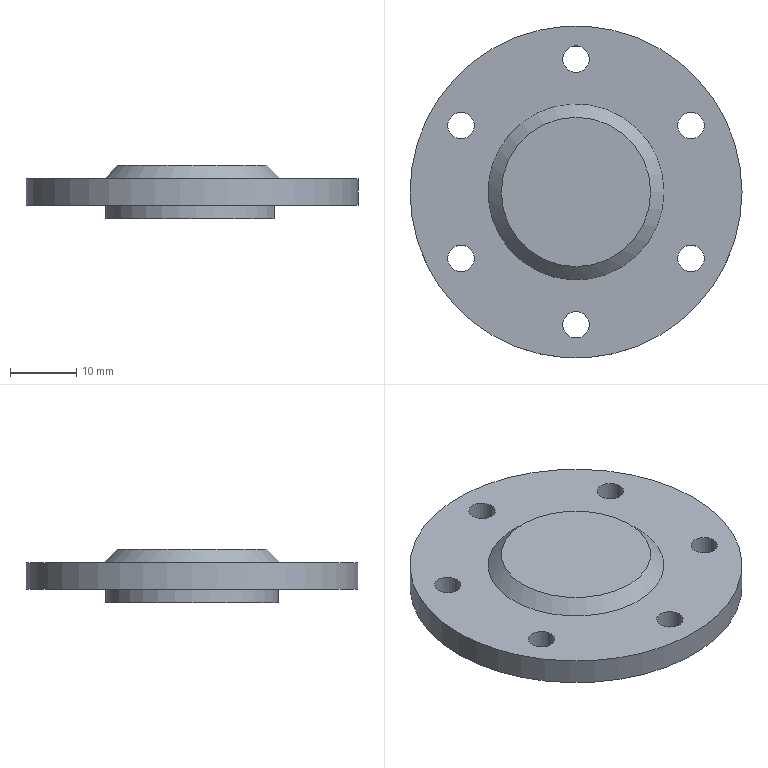Component | NX | 06__27 | 1 solid | 14 faces | box 50 x 50 x 8 mm | volume 9512 mm3 | cylinder 9 | plane 4 | cone 1 | commonest cylinder face diameters 4 x6 50 x1 26 x1 8 x1
STEP:
#1=CARTESIAN_POINT('',(0.,0.,0.));
#2=DIRECTION('',(0.,0.,1.));
#3=DIRECTION('',(1.,0.,0.));
#4=AXIS2_PLACEMENT_3D('',#1,#2,#3);
#5=CARTESIAN_POINT('',(28.272,109.608,238.432));
#6=VERTEX_POINT('',#5);
#7=CARTESIAN_POINT('',(17.022,109.608,238.432));
#8=DIRECTION('',(-0.,0.,1.));
#9=DIRECTION('',(1.,0.,0.));
#10=AXIS2_PLACEMENT_3D('',#7,#8,#9);
#11=CIRCLE('',#10,11.25);
#12=CARTESIAN_POINT('',(17.022,109.608,238.432));
#13=DIRECTION('',(-0.,0.,1.));
#14=DIRECTION('',(1.,0.,0.));
#15=AXIS2_PLACEMENT_3D('',#12,#13,#14);
#16=PLANE('',#15);
#17=CARTESIAN_POINT('',(0.,0.));
#18=DIRECTION('',(1.,0.));
#19=AXIS2_PLACEMENT_2D('',#17,#18);
#20=CIRCLE('',#19,11.25);
#21=(GEOMETRIC_REPRESENTATION_CONTEXT(2)PARAMETRIC_REPRESENTATION_CONTEXT()REPRESENTATION_CONTEXT('',''));
#22=DEFINITIONAL_REPRESENTATION('',(#20),#21);
#23=PCURVE('',#16,#22);
#24=CARTESIAN_POINT('',(17.022,109.608,238.432));
#25=DIRECTION('',(0.,0.,-1.));
#26=DIRECTION('',(-1.,0.,-0.));
#27=AXIS2_PLACEMENT_3D('',#24,#25,#26);
#28=CONICAL_SURFACE('',#27,11.25,0.7854);
#29=CARTESIAN_POINT('',(9.425,0.));
#30=DIRECTION('',(-1.,0.));
#31=VECTOR('',#30,1.);
#32=LINE('',#29,#31);
#33=(GEOMETRIC_REPRESENTATION_CONTEXT(2)PARAMETRIC_REPRESENTATION_CONTEXT()REPRESENTATION_CONTEXT('',''));
#34=DEFINITIONAL_REPRESENTATION('',(#32),#33);
#35=PCURVE('',#28,#34);
#36=SURFACE_CURVE('',#11,(#23,#35),.PCURVE_S1.);
#37=EDGE_CURVE('',#6,#6,#36,.T.);
#38=ORIENTED_EDGE('',*,*,#37,.T.);
#39=EDGE_LOOP('',(#38));
#40=FACE_BOUND('',#39,.T.);
#41=ADVANCED_FACE('',(#40),#16,.T.);
#42=CARTESIAN_POINT('',(30.272,109.608,236.432));
#43=VERTEX_POINT('',#42);
#44=CARTESIAN_POINT('',(17.022,109.608,236.432));
#45=DIRECTION('',(-0.,0.,1.));
#46=DIRECTION('',(1.,0.,0.));
#47=AXIS2_PLACEMENT_3D('',#44,#45,#46);
#48=CIRCLE('',#47,13.25);
#49=CARTESIAN_POINT('',(9.425,2.));
#50=DIRECTION('',(-1.,0.));
#51=VECTOR('',#50,1.);
#52=LINE('',#49,#51);
#53=(GEOMETRIC_REPRESENTATION_CONTEXT(2)PARAMETRIC_REPRESENTATION_CONTEXT()REPRESENTATION_CONTEXT('',''));
#54=DEFINITIONAL_REPRESENTATION('',(#52),#53);
#55=PCURVE('',#28,#54);
#56=CARTESIAN_POINT('',(30.272,109.608,236.432));
#57=DIRECTION('',(-0.,0.,1.));
#58=DIRECTION('',(1.,0.,0.));
#59=AXIS2_PLACEMENT_3D('',#56,#57,#58);
#60=PLANE('',#59);
#61=CARTESIAN_POINT('',(-13.25,0.));
#62=DIRECTION('',(1.,0.));
#63=AXIS2_PLACEMENT_2D('',#61,#62);
#64=CIRCLE('',#63,13.25);
#65=(GEOMETRIC_REPRESENTATION_CONTEXT(2)PARAMETRIC_REPRESENTATION_CONTEXT()REPRESENTATION_CONTEXT('',''));
#66=DEFINITIONAL_REPRESENTATION('',(#64),#65);
#67=PCURVE('',#60,#66);
#68=SURFACE_CURVE('',#48,(#55,#67),.PCURVE_S1.);
#69=EDGE_CURVE('',#43,#43,#68,.T.);
#70=ORIENTED_EDGE('',*,*,#69,.T.);
#71=CARTESIAN_POINT('',(28.272,109.608,238.432));
#72=CARTESIAN_POINT('',(30.272,109.608,236.432));
#73=B_SPLINE_CURVE_WITH_KNOTS('',1,(#71,#72),.UNSPECIFIED.,.F.,.F.,(2,2),(0.,2.828),.PIECEWISE_BEZIER_KNOTS.);
#74=CARTESIAN_POINT('',(3.142,0.));
#75=DIRECTION('',(0.,1.));
#76=VECTOR('',#75,1.);
#77=LINE('',#74,#76);
#78=(GEOMETRIC_REPRESENTATION_CONTEXT(2)PARAMETRIC_REPRESENTATION_CONTEXT()REPRESENTATION_CONTEXT('',''));
#79=DEFINITIONAL_REPRESENTATION('',(#77),#78);
#80=PCURVE('',#28,#79);
#81=CARTESIAN_POINT('',(9.425,0.));
#82=DIRECTION('',(0.,1.));
#83=VECTOR('',#82,1.);
#84=LINE('',#81,#83);
#85=(GEOMETRIC_REPRESENTATION_CONTEXT(2)PARAMETRIC_REPRESENTATION_CONTEXT()REPRESENTATION_CONTEXT('',''));
#86=DEFINITIONAL_REPRESENTATION('',(#84),#85);
#87=PCURVE('',#28,#86);
#88=SEAM_CURVE('',#73,(#80,#87),.PCURVE_S1.);
#89=EDGE_CURVE('',#6,#43,#88,.T.);
#90=ORIENTED_EDGE('',*,*,#89,.F.);
#91=ORIENTED_EDGE('',*,*,#37,.F.);
#92=ORIENTED_EDGE('',*,*,#89,.T.);
#93=EDGE_LOOP('',(#70,#90,#91,#92));
#94=FACE_BOUND('',#93,.T.);
#95=ADVANCED_FACE('',(#94),#28,.T.);
#96=CARTESIAN_POINT('',(19.022,129.608,236.432));
#97=VERTEX_POINT('',#96);
#98=CARTESIAN_POINT('',(17.022,129.608,236.432));
#99=DIRECTION('',(-0.,0.,1.));
#100=DIRECTION('',(1.,0.,0.));
#101=AXIS2_PLACEMENT_3D('',#98,#99,#100);
#102=CIRCLE('',#101,2.);
#103=CARTESIAN_POINT('',(-13.25,20.));
#104=DIRECTION('',(1.,0.));
#105=AXIS2_PLACEMENT_2D('',#103,#104);
#106=CIRCLE('',#105,2.);
#107=(GEOMETRIC_REPRESENTATION_CONTEXT(2)PARAMETRIC_REPRESENTATION_CONTEXT()REPRESENTATION_CONTEXT('',''));
#108=DEFINITIONAL_REPRESENTATION('',(#106),#107);
#109=PCURVE('',#60,#108);
#110=CARTESIAN_POINT('',(17.022,129.608,248.732));
#111=DIRECTION('',(0.,0.,-1.));
#112=DIRECTION('',(0.,1.,0.));
#113=AXIS2_PLACEMENT_3D('',#110,#111,#112);
#114=CYLINDRICAL_SURFACE('',#113,2.);
#115=CARTESIAN_POINT('',(7.854,12.3));
#116=DIRECTION('',(-1.,0.));
#117=VECTOR('',#116,1.);
#118=LINE('',#115,#117);
#119=(GEOMETRIC_REPRESENTATION_CONTEXT(2)PARAMETRIC_REPRESENTATION_CONTEXT()REPRESENTATION_CONTEXT('',''));
#120=DEFINITIONAL_REPRESENTATION('',(#118),#119);
#121=PCURVE('',#114,#120);
#122=SURFACE_CURVE('',#102,(#109,#121),.PCURVE_S1.);
#123=EDGE_CURVE('',#97,#97,#122,.T.);
#124=ORIENTED_EDGE('',*,*,#123,.F.);
#125=EDGE_LOOP('',(#124));
#126=FACE_BOUND('',#125,.T.);
#127=CARTESIAN_POINT('',(36.343,119.608,236.432));
#128=VERTEX_POINT('',#127);
#129=CARTESIAN_POINT('',(34.343,119.608,236.432));
#130=DIRECTION('',(-0.,0.,1.));
#131=DIRECTION('',(1.,0.,0.));
#132=AXIS2_PLACEMENT_3D('',#129,#130,#131);
#133=CIRCLE('',#132,2.);
#134=CARTESIAN_POINT('',(4.071,10.));
#135=DIRECTION('',(1.,0.));
#136=AXIS2_PLACEMENT_2D('',#134,#135);
#137=CIRCLE('',#136,2.);
#138=(GEOMETRIC_REPRESENTATION_CONTEXT(2)PARAMETRIC_REPRESENTATION_CONTEXT()REPRESENTATION_CONTEXT('',''));
#139=DEFINITIONAL_REPRESENTATION('',(#137),#138);
#140=PCURVE('',#60,#139);
#141=CARTESIAN_POINT('',(34.343,119.608,248.732));
#142=DIRECTION('',(0.,0.,-1.));
#143=DIRECTION('',(0.,1.,0.));
#144=AXIS2_PLACEMENT_3D('',#141,#142,#143);
#145=CYLINDRICAL_SURFACE('',#144,2.);
#146=CARTESIAN_POINT('',(7.854,12.3));
#147=DIRECTION('',(-1.,0.));
#148=VECTOR('',#147,1.);
#149=LINE('',#146,#148);
#150=(GEOMETRIC_REPRESENTATION_CONTEXT(2)PARAMETRIC_REPRESENTATION_CONTEXT()REPRESENTATION_CONTEXT('',''));
#151=DEFINITIONAL_REPRESENTATION('',(#149),#150);
#152=PCURVE('',#145,#151);
#153=SURFACE_CURVE('',#133,(#140,#152),.PCURVE_S1.);
#154=EDGE_CURVE('',#128,#128,#153,.T.);
#155=ORIENTED_EDGE('',*,*,#154,.F.);
#156=EDGE_LOOP('',(#155));
#157=FACE_BOUND('',#156,.T.);
#158=CARTESIAN_POINT('',(1.702,119.608,236.432));
#159=VERTEX_POINT('',#158);
#160=CARTESIAN_POINT('',(-0.2984,119.608,236.432));
#161=DIRECTION('',(-0.,0.,1.));
#162=DIRECTION('',(1.,0.,0.));
#163=AXIS2_PLACEMENT_3D('',#160,#161,#162);
#164=CIRCLE('',#163,2.);
#165=CARTESIAN_POINT('',(-30.571,10.));
#166=DIRECTION('',(1.,0.));
#167=AXIS2_PLACEMENT_2D('',#165,#166);
#168=CIRCLE('',#167,2.);
#169=(GEOMETRIC_REPRESENTATION_CONTEXT(2)PARAMETRIC_REPRESENTATION_CONTEXT()REPRESENTATION_CONTEXT('',''));
#170=DEFINITIONAL_REPRESENTATION('',(#168),#169);
#171=PCURVE('',#60,#170);
#172=CARTESIAN_POINT('',(-0.2984,119.608,248.732));
#173=DIRECTION('',(0.,0.,-1.));
#174=DIRECTION('',(0.,1.,0.));
#175=AXIS2_PLACEMENT_3D('',#172,#173,#174);
#176=CYLINDRICAL_SURFACE('',#175,2.);
#177=CARTESIAN_POINT('',(7.854,12.3));
#178=DIRECTION('',(-1.,0.));
#179=VECTOR('',#178,1.);
#180=LINE('',#177,#179);
#181=(GEOMETRIC_REPRESENTATION_CONTEXT(2)PARAMETRIC_REPRESENTATION_CONTEXT()REPRESENTATION_CONTEXT('',''));
#182=DEFINITIONAL_REPRESENTATION('',(#180),#181);
#183=PCURVE('',#176,#182);
#184=SURFACE_CURVE('',#164,(#171,#183),.PCURVE_S1.);
#185=EDGE_CURVE('',#159,#159,#184,.T.);
#186=ORIENTED_EDGE('',*,*,#185,.F.);
#187=EDGE_LOOP('',(#186));
#188=FACE_BOUND('',#187,.T.);
#189=CARTESIAN_POINT('',(36.343,99.608,236.432));
#190=VERTEX_POINT('',#189);
#191=CARTESIAN_POINT('',(34.343,99.608,236.432));
#192=DIRECTION('',(-0.,0.,1.));
#193=DIRECTION('',(1.,0.,0.));
#194=AXIS2_PLACEMENT_3D('',#191,#192,#193);
#195=CIRCLE('',#194,2.);
#196=CARTESIAN_POINT('',(4.071,-10.));
#197=DIRECTION('',(1.,0.));
#198=AXIS2_PLACEMENT_2D('',#196,#197);
#199=CIRCLE('',#198,2.);
#200=(GEOMETRIC_REPRESENTATION_CONTEXT(2)PARAMETRIC_REPRESENTATION_CONTEXT()REPRESENTATION_CONTEXT('',''));
#201=DEFINITIONAL_REPRESENTATION('',(#199),#200);
#202=PCURVE('',#60,#201);
#203=CARTESIAN_POINT('',(34.343,99.608,248.732));
#204=DIRECTION('',(0.,0.,-1.));
#205=DIRECTION('',(0.,1.,0.));
#206=AXIS2_PLACEMENT_3D('',#203,#204,#205);
#207=CYLINDRICAL_SURFACE('',#206,2.);
#208=CARTESIAN_POINT('',(7.854,12.3));
#209=DIRECTION('',(-1.,0.));
#210=VECTOR('',#209,1.);
#211=LINE('',#208,#210);
#212=(GEOMETRIC_REPRESENTATION_CONTEXT(2)PARAMETRIC_REPRESENTATION_CONTEXT()REPRESENTATION_CONTEXT('',''));
#213=DEFINITIONAL_REPRESENTATION('',(#211),#212);
#214=PCURVE('',#207,#213);
#215=SURFACE_CURVE('',#195,(#202,#214),.PCURVE_S1.);
#216=EDGE_CURVE('',#190,#190,#215,.T.);
#217=ORIENTED_EDGE('',*,*,#216,.F.);
#218=EDGE_LOOP('',(#217));
#219=FACE_BOUND('',#218,.T.);
#220=CARTESIAN_POINT('',(1.702,99.608,236.432));
#221=VERTEX_POINT('',#220);
#222=CARTESIAN_POINT('',(-0.2984,99.608,236.432));
#223=DIRECTION('',(-0.,0.,1.));
#224=DIRECTION('',(1.,0.,0.));
#225=AXIS2_PLACEMENT_3D('',#222,#223,#224);
#226=CIRCLE('',#225,2.);
#227=CARTESIAN_POINT('',(-30.571,-10.));
#228=DIRECTION('',(1.,0.));
#229=AXIS2_PLACEMENT_2D('',#227,#228);
#230=CIRCLE('',#229,2.);
#231=(GEOMETRIC_REPRESENTATION_CONTEXT(2)PARAMETRIC_REPRESENTATION_CONTEXT()REPRESENTATION_CONTEXT('',''));
#232=DEFINITIONAL_REPRESENTATION('',(#230),#231);
#233=PCURVE('',#60,#232);
#234=CARTESIAN_POINT('',(-0.2984,99.608,248.732));
#235=DIRECTION('',(0.,0.,-1.));
#236=DIRECTION('',(0.,1.,0.));
#237=AXIS2_PLACEMENT_3D('',#234,#235,#236);
#238=CYLINDRICAL_SURFACE('',#237,2.);
#239=CARTESIAN_POINT('',(7.854,12.3));
#240=DIRECTION('',(-1.,0.));
#241=VECTOR('',#240,1.);
#242=LINE('',#239,#241);
#243=(GEOMETRIC_REPRESENTATION_CONTEXT(2)PARAMETRIC_REPRESENTATION_CONTEXT()REPRESENTATION_CONTEXT('',''));
#244=DEFINITIONAL_REPRESENTATION('',(#242),#243);
#245=PCURVE('',#238,#244);
#246=SURFACE_CURVE('',#226,(#233,#245),.PCURVE_S1.);
#247=EDGE_CURVE('',#221,#221,#246,.T.);
#248=ORIENTED_EDGE('',*,*,#247,.F.);
#249=EDGE_LOOP('',(#248));
#250=FACE_BOUND('',#249,.T.);
#251=CARTESIAN_POINT('',(19.022,89.608,236.432));
#252=VERTEX_POINT('',#251);
#253=CARTESIAN_POINT('',(17.022,89.608,236.432));
#254=DIRECTION('',(-0.,0.,1.));
#255=DIRECTION('',(1.,0.,0.));
#256=AXIS2_PLACEMENT_3D('',#253,#254,#255);
#257=CIRCLE('',#256,2.);
#258=CARTESIAN_POINT('',(-13.25,-20.));
#259=DIRECTION('',(1.,0.));
#260=AXIS2_PLACEMENT_2D('',#258,#259);
#261=CIRCLE('',#260,2.);
#262=(GEOMETRIC_REPRESENTATION_CONTEXT(2)PARAMETRIC_REPRESENTATION_CONTEXT()REPRESENTATION_CONTEXT('',''));
#263=DEFINITIONAL_REPRESENTATION('',(#261),#262);
#264=PCURVE('',#60,#263);
#265=CARTESIAN_POINT('',(17.022,89.608,248.732));
#266=DIRECTION('',(0.,0.,-1.));
#267=DIRECTION('',(0.,1.,0.));
#268=AXIS2_PLACEMENT_3D('',#265,#266,#267);
#269=CYLINDRICAL_SURFACE('',#268,2.);
#270=CARTESIAN_POINT('',(7.854,12.3));
#271=DIRECTION('',(-1.,0.));
#272=VECTOR('',#271,1.);
#273=LINE('',#270,#272);
#274=(GEOMETRIC_REPRESENTATION_CONTEXT(2)PARAMETRIC_REPRESENTATION_CONTEXT()REPRESENTATION_CONTEXT('',''));
#275=DEFINITIONAL_REPRESENTATION('',(#273),#274);
#276=PCURVE('',#269,#275);
#277=SURFACE_CURVE('',#257,(#264,#276),.PCURVE_S1.);
#278=EDGE_CURVE('',#252,#252,#277,.T.);
#279=ORIENTED_EDGE('',*,*,#278,.F.);
#280=EDGE_LOOP('',(#279));
#281=FACE_BOUND('',#280,.T.);
#282=CARTESIAN_POINT('',(42.022,109.608,236.432));
#283=VERTEX_POINT('',#282);
#284=CARTESIAN_POINT('',(17.022,109.608,236.432));
#285=DIRECTION('',(-0.,0.,1.));
#286=DIRECTION('',(1.,0.,0.));
#287=AXIS2_PLACEMENT_3D('',#284,#285,#286);
#288=CIRCLE('',#287,25.);
#289=CARTESIAN_POINT('',(-13.25,0.));
#290=DIRECTION('',(1.,0.));
#291=AXIS2_PLACEMENT_2D('',#289,#290);
#292=CIRCLE('',#291,25.);
#293=(GEOMETRIC_REPRESENTATION_CONTEXT(2)PARAMETRIC_REPRESENTATION_CONTEXT()REPRESENTATION_CONTEXT('',''));
#294=DEFINITIONAL_REPRESENTATION('',(#292),#293);
#295=PCURVE('',#60,#294);
#296=CARTESIAN_POINT('',(17.022,109.608,230.432));
#297=DIRECTION('',(-0.,0.,1.));
#298=DIRECTION('',(1.,0.,0.));
#299=AXIS2_PLACEMENT_3D('',#296,#297,#298);
#300=CYLINDRICAL_SURFACE('',#299,25.);
#301=CARTESIAN_POINT('',(0.,6.));
#302=DIRECTION('',(1.,0.));
#303=VECTOR('',#302,1.);
#304=LINE('',#301,#303);
#305=(GEOMETRIC_REPRESENTATION_CONTEXT(2)PARAMETRIC_REPRESENTATION_CONTEXT()REPRESENTATION_CONTEXT('',''));
#306=DEFINITIONAL_REPRESENTATION('',(#304),#305);
#307=PCURVE('',#300,#306);
#308=SURFACE_CURVE('',#288,(#295,#307),.PCURVE_S1.);
#309=EDGE_CURVE('',#283,#283,#308,.T.);
#310=ORIENTED_EDGE('',*,*,#309,.T.);
#311=EDGE_LOOP('',(#310));
#312=FACE_BOUND('',#311,.T.);
#313=ORIENTED_EDGE('',*,*,#69,.F.);
#314=EDGE_LOOP('',(#313));
#315=FACE_BOUND('',#314,.T.);
#316=ADVANCED_FACE('',(#126,#157,#188,#219,#250,#281,#312,#315),#60,.T.);
#317=CARTESIAN_POINT('',(42.022,109.608,232.432));
#318=VERTEX_POINT('',#317);
#319=CARTESIAN_POINT('',(17.022,109.608,232.432));
#320=DIRECTION('',(-0.,0.,1.));
#321=DIRECTION('',(1.,0.,0.));
#322=AXIS2_PLACEMENT_3D('',#319,#320,#321);
#323=CIRCLE('',#322,25.);
#324=CARTESIAN_POINT('',(0.,2.));
#325=DIRECTION('',(1.,0.));
#326=VECTOR('',#325,1.);
#327=LINE('',#324,#326);
#328=(GEOMETRIC_REPRESENTATION_CONTEXT(2)PARAMETRIC_REPRESENTATION_CONTEXT()REPRESENTATION_CONTEXT('',''));
#329=DEFINITIONAL_REPRESENTATION('',(#327),#328);
#330=PCURVE('',#300,#329);
#331=CARTESIAN_POINT('',(42.022,109.608,232.432));
#332=DIRECTION('',(0.,0.,-1.));
#333=DIRECTION('',(-1.,0.,-0.));
#334=AXIS2_PLACEMENT_3D('',#331,#332,#333);
#335=PLANE('',#334);
#336=CARTESIAN_POINT('',(0.,0.));
#337=CARTESIAN_POINT('',(0.,43.301));
#338=CARTESIAN_POINT('',(37.5,21.651));
#339=CARTESIAN_POINT('',(75.,0.));
#340=CARTESIAN_POINT('',(37.5,-21.651));
#341=CARTESIAN_POINT('',(0.,-43.301));
#342=CARTESIAN_POINT('',(0.,0.));
#343=(BOUNDED_CURVE()B_SPLINE_CURVE(2,(#336,#337,#338,#339,#340,#341,#342),.UNSPECIFIED.,.T.,.F.)B_SPLINE_CURVE_WITH_KNOTS((1,2,2,2,2,1),(-2.094,0.,2.094,4.189,6.283,8.378),.UNSPECIFIED.)CURVE()GEOMETRIC_REPRESENTATION_ITEM()RATIONAL_B_SPLINE_CURVE((1.,0.5,1.,0.5,1.,0.5,1.))REPRESENTATION_ITEM(''));
#344=(GEOMETRIC_REPRESENTATION_CONTEXT(2)PARAMETRIC_REPRESENTATION_CONTEXT()REPRESENTATION_CONTEXT('',''));
#345=DEFINITIONAL_REPRESENTATION('',(#343),#344);
#346=PCURVE('',#335,#345);
#347=SURFACE_CURVE('',#323,(#330,#346),.PCURVE_S1.);
#348=EDGE_CURVE('',#318,#318,#347,.T.);
#349=ORIENTED_EDGE('',*,*,#348,.T.);
#350=CARTESIAN_POINT('',(42.022,109.608,232.432));
#351=CARTESIAN_POINT('',(42.022,109.608,236.432));
#352=B_SPLINE_CURVE_WITH_KNOTS('',1,(#350,#351),.UNSPECIFIED.,.F.,.F.,(2,2),(2.,6.),.PIECEWISE_BEZIER_KNOTS.);
#353=CARTESIAN_POINT('',(6.283,0.));
#354=DIRECTION('',(0.,1.));
#355=VECTOR('',#354,1.);
#356=LINE('',#353,#355);
#357=(GEOMETRIC_REPRESENTATION_CONTEXT(2)PARAMETRIC_REPRESENTATION_CONTEXT()REPRESENTATION_CONTEXT('',''));
#358=DEFINITIONAL_REPRESENTATION('',(#356),#357);
#359=PCURVE('',#300,#358);
#360=CARTESIAN_POINT('',(0.,0.));
#361=DIRECTION('',(0.,1.));
#362=VECTOR('',#361,1.);
#363=LINE('',#360,#362);
#364=(GEOMETRIC_REPRESENTATION_CONTEXT(2)PARAMETRIC_REPRESENTATION_CONTEXT()REPRESENTATION_CONTEXT('',''));
#365=DEFINITIONAL_REPRESENTATION('',(#363),#364);
#366=PCURVE('',#300,#365);
#367=SEAM_CURVE('',#352,(#359,#366),.PCURVE_S1.);
#368=EDGE_CURVE('',#318,#283,#367,.T.);
#369=ORIENTED_EDGE('',*,*,#368,.T.);
#370=ORIENTED_EDGE('',*,*,#309,.F.);
#371=ORIENTED_EDGE('',*,*,#368,.F.);
#372=EDGE_LOOP('',(#349,#369,#370,#371));
#373=FACE_BOUND('',#372,.T.);
#374=ADVANCED_FACE('',(#373),#300,.T.);
#375=CARTESIAN_POINT('',(29.407,113.56,232.432));
#376=VERTEX_POINT('',#375);
#377=CARTESIAN_POINT('',(29.407,105.656,232.432));
#378=VERTEX_POINT('',#377);
#379=CARTESIAN_POINT('',(17.022,109.608,232.432));
#380=DIRECTION('',(-0.,0.,1.));
#381=DIRECTION('',(1.,0.,0.));
#382=AXIS2_PLACEMENT_3D('',#379,#380,#381);
#383=CIRCLE('',#382,13.);
#384=CARTESIAN_POINT('',(12.,0.));
#385=CARTESIAN_POINT('',(12.,22.517));
#386=CARTESIAN_POINT('',(31.5,11.258));
#387=CARTESIAN_POINT('',(51.,0.));
#388=CARTESIAN_POINT('',(31.5,-11.258));
#389=CARTESIAN_POINT('',(12.,-22.517));
#390=CARTESIAN_POINT('',(12.,0.));
#391=(BOUNDED_CURVE()B_SPLINE_CURVE(2,(#384,#385,#386,#387,#388,#389,#390),.UNSPECIFIED.,.T.,.F.)B_SPLINE_CURVE_WITH_KNOTS((1,2,2,2,2,1),(-2.094,0.,2.094,4.189,6.283,8.378),.UNSPECIFIED.)CURVE()GEOMETRIC_REPRESENTATION_ITEM()RATIONAL_B_SPLINE_CURVE((1.,0.5,1.,0.5,1.,0.5,1.))REPRESENTATION_ITEM(''));
#392=(GEOMETRIC_REPRESENTATION_CONTEXT(2)PARAMETRIC_REPRESENTATION_CONTEXT()REPRESENTATION_CONTEXT('',''));
#393=DEFINITIONAL_REPRESENTATION('',(#391),#392);
#394=PCURVE('',#335,#393);
#395=CARTESIAN_POINT('',(17.022,109.608,230.432));
#396=DIRECTION('',(-0.,0.,1.));
#397=DIRECTION('',(1.,0.,0.));
#398=AXIS2_PLACEMENT_3D('',#395,#396,#397);
#399=CYLINDRICAL_SURFACE('',#398,13.);
#400=CARTESIAN_POINT('',(-0.,2.));
#401=DIRECTION('',(1.,0.));
#402=VECTOR('',#401,1.);
#403=LINE('',#400,#402);
#404=(GEOMETRIC_REPRESENTATION_CONTEXT(2)PARAMETRIC_REPRESENTATION_CONTEXT()REPRESENTATION_CONTEXT('',''));
#405=DEFINITIONAL_REPRESENTATION('',(#403),#404);
#406=PCURVE('',#399,#405);
#407=SURFACE_CURVE('',#383,(#394,#406),.PCURVE_S1.);
#408=EDGE_CURVE('',#376,#378,#407,.T.);
#409=ORIENTED_EDGE('',*,*,#408,.T.);
#410=CARTESIAN_POINT('',(30.022,109.608,232.432));
#411=DIRECTION('',(0.,0.,-1.));
#412=DIRECTION('',(0.,1.,0.));
#413=AXIS2_PLACEMENT_3D('',#410,#411,#412);
#414=CIRCLE('',#413,4.);
#415=CARTESIAN_POINT('',(12.,0.));
#416=DIRECTION('',(0.,1.));
#417=AXIS2_PLACEMENT_2D('',#415,#416);
#418=CIRCLE('',#417,4.);
#419=(GEOMETRIC_REPRESENTATION_CONTEXT(2)PARAMETRIC_REPRESENTATION_CONTEXT()REPRESENTATION_CONTEXT('',''));
#420=DEFINITIONAL_REPRESENTATION('',(#418),#419);
#421=PCURVE('',#335,#420);
#422=CARTESIAN_POINT('',(30.022,109.608,232.432));
#423=DIRECTION('',(0.,0.,-1.));
#424=DIRECTION('',(0.,1.,0.));
#425=AXIS2_PLACEMENT_3D('',#422,#423,#424);
#426=CYLINDRICAL_SURFACE('',#425,4.);
#427=CARTESIAN_POINT('',(-0.,0.));
#428=DIRECTION('',(1.,0.));
#429=VECTOR('',#428,1.);
#430=LINE('',#427,#429);
#431=(GEOMETRIC_REPRESENTATION_CONTEXT(2)PARAMETRIC_REPRESENTATION_CONTEXT()REPRESENTATION_CONTEXT('',''));
#432=DEFINITIONAL_REPRESENTATION('',(#430),#431);
#433=PCURVE('',#426,#432);
#434=SURFACE_CURVE('',#414,(#421,#433),.PCURVE_S1.);
#435=EDGE_CURVE('',#378,#376,#434,.T.);
#436=ORIENTED_EDGE('',*,*,#435,.T.);
#437=EDGE_LOOP('',(#409,#436));
#438=FACE_BOUND('',#437,.T.);
#439=CARTESIAN_POINT('',(15.022,129.608,232.432));
#440=VERTEX_POINT('',#439);
#441=CARTESIAN_POINT('',(19.022,129.608,232.432));
#442=VERTEX_POINT('',#441);
#443=CARTESIAN_POINT('',(17.022,129.608,232.432));
#444=DIRECTION('',(0.,0.,-1.));
#445=DIRECTION('',(-1.,0.,-0.));
#446=AXIS2_PLACEMENT_3D('',#443,#444,#445);
#447=CIRCLE('',#446,2.);
#448=CARTESIAN_POINT('',(25.,20.));
#449=DIRECTION('',(1.,0.));
#450=AXIS2_PLACEMENT_2D('',#448,#449);
#451=CIRCLE('',#450,2.);
#452=(GEOMETRIC_REPRESENTATION_CONTEXT(2)PARAMETRIC_REPRESENTATION_CONTEXT()REPRESENTATION_CONTEXT('',''));
#453=DEFINITIONAL_REPRESENTATION('',(#451),#452);
#454=PCURVE('',#335,#453);
#455=CARTESIAN_POINT('',(4.712,16.3));
#456=DIRECTION('',(1.,0.));
#457=VECTOR('',#456,1.);
#458=LINE('',#455,#457);
#459=(GEOMETRIC_REPRESENTATION_CONTEXT(2)PARAMETRIC_REPRESENTATION_CONTEXT()REPRESENTATION_CONTEXT('',''));
#460=DEFINITIONAL_REPRESENTATION('',(#458),#459);
#461=PCURVE('',#114,#460);
#462=SURFACE_CURVE('',#447,(#454,#461),.PCURVE_S1.);
#463=EDGE_CURVE('',#440,#442,#462,.T.);
#464=ORIENTED_EDGE('',*,*,#463,.F.);
#465=CARTESIAN_POINT('',(17.022,129.608,232.432));
#466=DIRECTION('',(0.,0.,-1.));
#467=DIRECTION('',(-1.,0.,-0.));
#468=AXIS2_PLACEMENT_3D('',#465,#466,#467);
#469=CIRCLE('',#468,2.);
#470=CARTESIAN_POINT('',(25.,20.));
#471=DIRECTION('',(1.,0.));
#472=AXIS2_PLACEMENT_2D('',#470,#471);
#473=CIRCLE('',#472,2.);
#474=(GEOMETRIC_REPRESENTATION_CONTEXT(2)PARAMETRIC_REPRESENTATION_CONTEXT()REPRESENTATION_CONTEXT('',''));
#475=DEFINITIONAL_REPRESENTATION('',(#473),#474);
#476=PCURVE('',#335,#475);
#477=CARTESIAN_POINT('',(-1.571,16.3));
#478=DIRECTION('',(1.,0.));
#479=VECTOR('',#478,1.);
#480=LINE('',#477,#479);
#481=(GEOMETRIC_REPRESENTATION_CONTEXT(2)PARAMETRIC_REPRESENTATION_CONTEXT()REPRESENTATION_CONTEXT('',''));
#482=DEFINITIONAL_REPRESENTATION('',(#480),#481);
#483=PCURVE('',#114,#482);
#484=SURFACE_CURVE('',#469,(#476,#483),.PCURVE_S1.);
#485=EDGE_CURVE('',#442,#440,#484,.T.);
#486=ORIENTED_EDGE('',*,*,#485,.F.);
#487=EDGE_LOOP('',(#464,#486));
#488=FACE_BOUND('',#487,.T.);
#489=CARTESIAN_POINT('',(32.343,119.608,232.432));
#490=VERTEX_POINT('',#489);
#491=CARTESIAN_POINT('',(36.343,119.608,232.432));
#492=VERTEX_POINT('',#491);
#493=CARTESIAN_POINT('',(34.343,119.608,232.432));
#494=DIRECTION('',(0.,0.,-1.));
#495=DIRECTION('',(-1.,0.,-0.));
#496=AXIS2_PLACEMENT_3D('',#493,#494,#495);
#497=CIRCLE('',#496,2.);
#498=CARTESIAN_POINT('',(7.679,10.));
#499=DIRECTION('',(1.,0.));
#500=AXIS2_PLACEMENT_2D('',#498,#499);
#501=CIRCLE('',#500,2.);
#502=(GEOMETRIC_REPRESENTATION_CONTEXT(2)PARAMETRIC_REPRESENTATION_CONTEXT()REPRESENTATION_CONTEXT('',''));
#503=DEFINITIONAL_REPRESENTATION('',(#501),#502);
#504=PCURVE('',#335,#503);
#505=CARTESIAN_POINT('',(4.712,16.3));
#506=DIRECTION('',(1.,0.));
#507=VECTOR('',#506,1.);
#508=LINE('',#505,#507);
#509=(GEOMETRIC_REPRESENTATION_CONTEXT(2)PARAMETRIC_REPRESENTATION_CONTEXT()REPRESENTATION_CONTEXT('',''));
#510=DEFINITIONAL_REPRESENTATION('',(#508),#509);
#511=PCURVE('',#145,#510);
#512=SURFACE_CURVE('',#497,(#504,#511),.PCURVE_S1.);
#513=EDGE_CURVE('',#490,#492,#512,.T.);
#514=ORIENTED_EDGE('',*,*,#513,.F.);
#515=CARTESIAN_POINT('',(34.343,119.608,232.432));
#516=DIRECTION('',(0.,0.,-1.));
#517=DIRECTION('',(-1.,0.,-0.));
#518=AXIS2_PLACEMENT_3D('',#515,#516,#517);
#519=CIRCLE('',#518,2.);
#520=CARTESIAN_POINT('',(7.679,10.));
#521=DIRECTION('',(1.,0.));
#522=AXIS2_PLACEMENT_2D('',#520,#521);
#523=CIRCLE('',#522,2.);
#524=(GEOMETRIC_REPRESENTATION_CONTEXT(2)PARAMETRIC_REPRESENTATION_CONTEXT()REPRESENTATION_CONTEXT('',''));
#525=DEFINITIONAL_REPRESENTATION('',(#523),#524);
#526=PCURVE('',#335,#525);
#527=CARTESIAN_POINT('',(-1.571,16.3));
#528=DIRECTION('',(1.,0.));
#529=VECTOR('',#528,1.);
#530=LINE('',#527,#529);
#531=(GEOMETRIC_REPRESENTATION_CONTEXT(2)PARAMETRIC_REPRESENTATION_CONTEXT()REPRESENTATION_CONTEXT('',''));
#532=DEFINITIONAL_REPRESENTATION('',(#530),#531);
#533=PCURVE('',#145,#532);
#534=SURFACE_CURVE('',#519,(#526,#533),.PCURVE_S1.);
#535=EDGE_CURVE('',#492,#490,#534,.T.);
#536=ORIENTED_EDGE('',*,*,#535,.F.);
#537=EDGE_LOOP('',(#514,#536));
#538=FACE_BOUND('',#537,.T.);
#539=CARTESIAN_POINT('',(-2.298,119.608,232.432));
#540=VERTEX_POINT('',#539);
#541=CARTESIAN_POINT('',(1.702,119.608,232.432));
#542=VERTEX_POINT('',#541);
#543=CARTESIAN_POINT('',(-0.2984,119.608,232.432));
#544=DIRECTION('',(0.,0.,-1.));
#545=DIRECTION('',(-1.,0.,-0.));
#546=AXIS2_PLACEMENT_3D('',#543,#544,#545);
#547=CIRCLE('',#546,2.);
#548=CARTESIAN_POINT('',(42.321,10.));
#549=DIRECTION('',(1.,0.));
#550=AXIS2_PLACEMENT_2D('',#548,#549);
#551=CIRCLE('',#550,2.);
#552=(GEOMETRIC_REPRESENTATION_CONTEXT(2)PARAMETRIC_REPRESENTATION_CONTEXT()REPRESENTATION_CONTEXT('',''));
#553=DEFINITIONAL_REPRESENTATION('',(#551),#552);
#554=PCURVE('',#335,#553);
#555=CARTESIAN_POINT('',(4.712,16.3));
#556=DIRECTION('',(1.,0.));
#557=VECTOR('',#556,1.);
#558=LINE('',#555,#557);
#559=(GEOMETRIC_REPRESENTATION_CONTEXT(2)PARAMETRIC_REPRESENTATION_CONTEXT()REPRESENTATION_CONTEXT('',''));
#560=DEFINITIONAL_REPRESENTATION('',(#558),#559);
#561=PCURVE('',#176,#560);
#562=SURFACE_CURVE('',#547,(#554,#561),.PCURVE_S1.);
#563=EDGE_CURVE('',#540,#542,#562,.T.);
#564=ORIENTED_EDGE('',*,*,#563,.F.);
#565=CARTESIAN_POINT('',(-0.2984,119.608,232.432));
#566=DIRECTION('',(0.,0.,-1.));
#567=DIRECTION('',(-1.,0.,-0.));
#568=AXIS2_PLACEMENT_3D('',#565,#566,#567);
#569=CIRCLE('',#568,2.);
#570=CARTESIAN_POINT('',(42.321,10.));
#571=DIRECTION('',(1.,0.));
#572=AXIS2_PLACEMENT_2D('',#570,#571);
#573=CIRCLE('',#572,2.);
#574=(GEOMETRIC_REPRESENTATION_CONTEXT(2)PARAMETRIC_REPRESENTATION_CONTEXT()REPRESENTATION_CONTEXT('',''));
#575=DEFINITIONAL_REPRESENTATION('',(#573),#574);
#576=PCURVE('',#335,#575);
#577=CARTESIAN_POINT('',(-1.571,16.3));
#578=DIRECTION('',(1.,0.));
#579=VECTOR('',#578,1.);
#580=LINE('',#577,#579);
#581=(GEOMETRIC_REPRESENTATION_CONTEXT(2)PARAMETRIC_REPRESENTATION_CONTEXT()REPRESENTATION_CONTEXT('',''));
#582=DEFINITIONAL_REPRESENTATION('',(#580),#581);
#583=PCURVE('',#176,#582);
#584=SURFACE_CURVE('',#569,(#576,#583),.PCURVE_S1.);
#585=EDGE_CURVE('',#542,#540,#584,.T.);
#586=ORIENTED_EDGE('',*,*,#585,.F.);
#587=EDGE_LOOP('',(#564,#586));
#588=FACE_BOUND('',#587,.T.);
#589=CARTESIAN_POINT('',(32.343,99.608,232.432));
#590=VERTEX_POINT('',#589);
#591=CARTESIAN_POINT('',(36.343,99.608,232.432));
#592=VERTEX_POINT('',#591);
#593=CARTESIAN_POINT('',(34.343,99.608,232.432));
#594=DIRECTION('',(0.,0.,-1.));
#595=DIRECTION('',(-1.,0.,-0.));
#596=AXIS2_PLACEMENT_3D('',#593,#594,#595);
#597=CIRCLE('',#596,2.);
#598=CARTESIAN_POINT('',(7.679,-10.));
#599=DIRECTION('',(1.,0.));
#600=AXIS2_PLACEMENT_2D('',#598,#599);
#601=CIRCLE('',#600,2.);
#602=(GEOMETRIC_REPRESENTATION_CONTEXT(2)PARAMETRIC_REPRESENTATION_CONTEXT()REPRESENTATION_CONTEXT('',''));
#603=DEFINITIONAL_REPRESENTATION('',(#601),#602);
#604=PCURVE('',#335,#603);
#605=CARTESIAN_POINT('',(4.712,16.3));
#606=DIRECTION('',(1.,0.));
#607=VECTOR('',#606,1.);
#608=LINE('',#605,#607);
#609=(GEOMETRIC_REPRESENTATION_CONTEXT(2)PARAMETRIC_REPRESENTATION_CONTEXT()REPRESENTATION_CONTEXT('',''));
#610=DEFINITIONAL_REPRESENTATION('',(#608),#609);
#611=PCURVE('',#207,#610);
#612=SURFACE_CURVE('',#597,(#604,#611),.PCURVE_S1.);
#613=EDGE_CURVE('',#590,#592,#612,.T.);
#614=ORIENTED_EDGE('',*,*,#613,.F.);
#615=CARTESIAN_POINT('',(34.343,99.608,232.432));
#616=DIRECTION('',(0.,0.,-1.));
#617=DIRECTION('',(-1.,0.,-0.));
#618=AXIS2_PLACEMENT_3D('',#615,#616,#617);
#619=CIRCLE('',#618,2.);
#620=CARTESIAN_POINT('',(7.679,-10.));
#621=DIRECTION('',(1.,0.));
#622=AXIS2_PLACEMENT_2D('',#620,#621);
#623=CIRCLE('',#622,2.);
#624=(GEOMETRIC_REPRESENTATION_CONTEXT(2)PARAMETRIC_REPRESENTATION_CONTEXT()REPRESENTATION_CONTEXT('',''));
#625=DEFINITIONAL_REPRESENTATION('',(#623),#624);
#626=PCURVE('',#335,#625);
#627=CARTESIAN_POINT('',(-1.571,16.3));
#628=DIRECTION('',(1.,0.));
#629=VECTOR('',#628,1.);
#630=LINE('',#627,#629);
#631=(GEOMETRIC_REPRESENTATION_CONTEXT(2)PARAMETRIC_REPRESENTATION_CONTEXT()REPRESENTATION_CONTEXT('',''));
#632=DEFINITIONAL_REPRESENTATION('',(#630),#631);
#633=PCURVE('',#207,#632);
#634=SURFACE_CURVE('',#619,(#626,#633),.PCURVE_S1.);
#635=EDGE_CURVE('',#592,#590,#634,.T.);
#636=ORIENTED_EDGE('',*,*,#635,.F.);
#637=EDGE_LOOP('',(#614,#636));
#638=FACE_BOUND('',#637,.T.);
#639=CARTESIAN_POINT('',(-2.298,99.608,232.432));
#640=VERTEX_POINT('',#639);
#641=CARTESIAN_POINT('',(1.702,99.608,232.432));
#642=VERTEX_POINT('',#641);
#643=CARTESIAN_POINT('',(-0.2984,99.608,232.432));
#644=DIRECTION('',(0.,0.,-1.));
#645=DIRECTION('',(-1.,0.,-0.));
#646=AXIS2_PLACEMENT_3D('',#643,#644,#645);
#647=CIRCLE('',#646,2.);
#648=CARTESIAN_POINT('',(42.321,-10.));
#649=DIRECTION('',(1.,0.));
#650=AXIS2_PLACEMENT_2D('',#648,#649);
#651=CIRCLE('',#650,2.);
#652=(GEOMETRIC_REPRESENTATION_CONTEXT(2)PARAMETRIC_REPRESENTATION_CONTEXT()REPRESENTATION_CONTEXT('',''));
#653=DEFINITIONAL_REPRESENTATION('',(#651),#652);
#654=PCURVE('',#335,#653);
#655=CARTESIAN_POINT('',(4.712,16.3));
#656=DIRECTION('',(1.,0.));
#657=VECTOR('',#656,1.);
#658=LINE('',#655,#657);
#659=(GEOMETRIC_REPRESENTATION_CONTEXT(2)PARAMETRIC_REPRESENTATION_CONTEXT()REPRESENTATION_CONTEXT('',''));
#660=DEFINITIONAL_REPRESENTATION('',(#658),#659);
#661=PCURVE('',#238,#660);
#662=SURFACE_CURVE('',#647,(#654,#661),.PCURVE_S1.);
#663=EDGE_CURVE('',#640,#642,#662,.T.);
#664=ORIENTED_EDGE('',*,*,#663,.F.);
#665=CARTESIAN_POINT('',(-0.2984,99.608,232.432));
#666=DIRECTION('',(0.,0.,-1.));
#667=DIRECTION('',(-1.,0.,-0.));
#668=AXIS2_PLACEMENT_3D('',#665,#666,#667);
#669=CIRCLE('',#668,2.);
#670=CARTESIAN_POINT('',(42.321,-10.));
#671=DIRECTION('',(1.,0.));
#672=AXIS2_PLACEMENT_2D('',#670,#671);
#673=CIRCLE('',#672,2.);
#674=(GEOMETRIC_REPRESENTATION_CONTEXT(2)PARAMETRIC_REPRESENTATION_CONTEXT()REPRESENTATION_CONTEXT('',''));
#675=DEFINITIONAL_REPRESENTATION('',(#673),#674);
#676=PCURVE('',#335,#675);
#677=CARTESIAN_POINT('',(-1.571,16.3));
#678=DIRECTION('',(1.,0.));
#679=VECTOR('',#678,1.);
#680=LINE('',#677,#679);
#681=(GEOMETRIC_REPRESENTATION_CONTEXT(2)PARAMETRIC_REPRESENTATION_CONTEXT()REPRESENTATION_CONTEXT('',''));
#682=DEFINITIONAL_REPRESENTATION('',(#680),#681);
#683=PCURVE('',#238,#682);
#684=SURFACE_CURVE('',#669,(#676,#683),.PCURVE_S1.);
#685=EDGE_CURVE('',#642,#640,#684,.T.);
#686=ORIENTED_EDGE('',*,*,#685,.F.);
#687=EDGE_LOOP('',(#664,#686));
#688=FACE_BOUND('',#687,.T.);
#689=CARTESIAN_POINT('',(15.022,89.608,232.432));
#690=VERTEX_POINT('',#689);
#691=CARTESIAN_POINT('',(19.022,89.608,232.432));
#692=VERTEX_POINT('',#691);
#693=CARTESIAN_POINT('',(17.022,89.608,232.432));
#694=DIRECTION('',(0.,0.,-1.));
#695=DIRECTION('',(-1.,0.,-0.));
#696=AXIS2_PLACEMENT_3D('',#693,#694,#695);
#697=CIRCLE('',#696,2.);
#698=CARTESIAN_POINT('',(25.,-20.));
#699=DIRECTION('',(1.,0.));
#700=AXIS2_PLACEMENT_2D('',#698,#699);
#701=CIRCLE('',#700,2.);
#702=(GEOMETRIC_REPRESENTATION_CONTEXT(2)PARAMETRIC_REPRESENTATION_CONTEXT()REPRESENTATION_CONTEXT('',''));
#703=DEFINITIONAL_REPRESENTATION('',(#701),#702);
#704=PCURVE('',#335,#703);
#705=CARTESIAN_POINT('',(4.712,16.3));
#706=DIRECTION('',(1.,0.));
#707=VECTOR('',#706,1.);
#708=LINE('',#705,#707);
#709=(GEOMETRIC_REPRESENTATION_CONTEXT(2)PARAMETRIC_REPRESENTATION_CONTEXT()REPRESENTATION_CONTEXT('',''));
#710=DEFINITIONAL_REPRESENTATION('',(#708),#709);
#711=PCURVE('',#269,#710);
#712=SURFACE_CURVE('',#697,(#704,#711),.PCURVE_S1.);
#713=EDGE_CURVE('',#690,#692,#712,.T.);
#714=ORIENTED_EDGE('',*,*,#713,.F.);
#715=CARTESIAN_POINT('',(17.022,89.608,232.432));
#716=DIRECTION('',(0.,0.,-1.));
#717=DIRECTION('',(-1.,0.,-0.));
#718=AXIS2_PLACEMENT_3D('',#715,#716,#717);
#719=CIRCLE('',#718,2.);
#720=CARTESIAN_POINT('',(25.,-20.));
#721=DIRECTION('',(1.,0.));
#722=AXIS2_PLACEMENT_2D('',#720,#721);
#723=CIRCLE('',#722,2.);
#724=(GEOMETRIC_REPRESENTATION_CONTEXT(2)PARAMETRIC_REPRESENTATION_CONTEXT()REPRESENTATION_CONTEXT('',''));
#725=DEFINITIONAL_REPRESENTATION('',(#723),#724);
#726=PCURVE('',#335,#725);
#727=CARTESIAN_POINT('',(-1.571,16.3));
#728=DIRECTION('',(1.,0.));
#729=VECTOR('',#728,1.);
#730=LINE('',#727,#729);
#731=(GEOMETRIC_REPRESENTATION_CONTEXT(2)PARAMETRIC_REPRESENTATION_CONTEXT()REPRESENTATION_CONTEXT('',''));
#732=DEFINITIONAL_REPRESENTATION('',(#730),#731);
#733=PCURVE('',#269,#732);
#734=SURFACE_CURVE('',#719,(#726,#733),.PCURVE_S1.);
#735=EDGE_CURVE('',#692,#690,#734,.T.);
#736=ORIENTED_EDGE('',*,*,#735,.F.);
#737=EDGE_LOOP('',(#714,#736));
#738=FACE_BOUND('',#737,.T.);
#739=ORIENTED_EDGE('',*,*,#348,.F.);
#740=EDGE_LOOP('',(#739));
#741=FACE_BOUND('',#740,.T.);
#742=ADVANCED_FACE('',(#438,#488,#538,#588,#638,#688,#738,#741),#335,.T.);
#743=CARTESIAN_POINT('',(29.407,113.56,230.432));
#744=VERTEX_POINT('',#743);
#745=CARTESIAN_POINT('',(29.407,113.56,231.432));
#746=DIRECTION('',(0.,0.,1.));
#747=VECTOR('',#746,1.);
#748=LINE('',#745,#747);
#749=CARTESIAN_POINT('',(0.3089,1.));
#750=DIRECTION('',(-0.,1.));
#751=VECTOR('',#750,1.);
#752=LINE('',#749,#751);
#753=(GEOMETRIC_REPRESENTATION_CONTEXT(2)PARAMETRIC_REPRESENTATION_CONTEXT()REPRESENTATION_CONTEXT('',''));
#754=DEFINITIONAL_REPRESENTATION('',(#752),#753);
#755=PCURVE('',#399,#754);
#756=CARTESIAN_POINT('',(6.129,1.));
#757=DIRECTION('',(0.,-1.));
#758=VECTOR('',#757,1.);
#759=LINE('',#756,#758);
#760=(GEOMETRIC_REPRESENTATION_CONTEXT(2)PARAMETRIC_REPRESENTATION_CONTEXT()REPRESENTATION_CONTEXT('',''));
#761=DEFINITIONAL_REPRESENTATION('',(#759),#760);
#762=PCURVE('',#426,#761);
#763=SURFACE_CURVE('',#748,(#755,#762),.PCURVE_S1.);
#764=EDGE_CURVE('',#744,#376,#763,.T.);
#765=ORIENTED_EDGE('',*,*,#764,.F.);
#766=CARTESIAN_POINT('',(29.407,105.656,230.432));
#767=VERTEX_POINT('',#766);
#768=CARTESIAN_POINT('',(17.022,109.608,230.432));
#769=DIRECTION('',(-0.,0.,1.));
#770=DIRECTION('',(1.,0.,0.));
#771=AXIS2_PLACEMENT_3D('',#768,#769,#770);
#772=CIRCLE('',#771,13.);
#773=CARTESIAN_POINT('',(-0.,0.));
#774=DIRECTION('',(1.,0.));
#775=VECTOR('',#774,1.);
#776=LINE('',#773,#775);
#777=(GEOMETRIC_REPRESENTATION_CONTEXT(2)PARAMETRIC_REPRESENTATION_CONTEXT()REPRESENTATION_CONTEXT('',''));
#778=DEFINITIONAL_REPRESENTATION('',(#776),#777);
#779=PCURVE('',#399,#778);
#780=CARTESIAN_POINT('',(30.022,109.608,230.432));
#781=DIRECTION('',(0.,0.,-1.));
#782=DIRECTION('',(-1.,0.,-0.));
#783=AXIS2_PLACEMENT_3D('',#780,#781,#782);
#784=PLANE('',#783);
#785=CARTESIAN_POINT('',(0.,0.));
#786=CARTESIAN_POINT('',(0.,22.517));
#787=CARTESIAN_POINT('',(19.5,11.258));
#788=CARTESIAN_POINT('',(39.,0.));
#789=CARTESIAN_POINT('',(19.5,-11.258));
#790=CARTESIAN_POINT('',(0.,-22.517));
#791=CARTESIAN_POINT('',(0.,0.));
#792=(BOUNDED_CURVE()B_SPLINE_CURVE(2,(#785,#786,#787,#788,#789,#790,#791),.UNSPECIFIED.,.T.,.F.)B_SPLINE_CURVE_WITH_KNOTS((1,2,2,2,2,1),(-2.094,0.,2.094,4.189,6.283,8.378),.UNSPECIFIED.)CURVE()GEOMETRIC_REPRESENTATION_ITEM()RATIONAL_B_SPLINE_CURVE((1.,0.5,1.,0.5,1.,0.5,1.))REPRESENTATION_ITEM(''));
#793=(GEOMETRIC_REPRESENTATION_CONTEXT(2)PARAMETRIC_REPRESENTATION_CONTEXT()REPRESENTATION_CONTEXT('',''));
#794=DEFINITIONAL_REPRESENTATION('',(#792),#793);
#795=PCURVE('',#784,#794);
#796=SURFACE_CURVE('',#772,(#779,#795),.PCURVE_S1.);
#797=EDGE_CURVE('',#744,#767,#796,.T.);
#798=ORIENTED_EDGE('',*,*,#797,.T.);
#799=CARTESIAN_POINT('',(29.407,105.656,231.432));
#800=DIRECTION('',(0.,0.,-1.));
#801=VECTOR('',#800,1.);
#802=LINE('',#799,#801);
#803=CARTESIAN_POINT('',(5.974,1.));
#804=DIRECTION('',(0.,-1.));
#805=VECTOR('',#804,1.);
#806=LINE('',#803,#805);
#807=(GEOMETRIC_REPRESENTATION_CONTEXT(2)PARAMETRIC_REPRESENTATION_CONTEXT()REPRESENTATION_CONTEXT('',''));
#808=DEFINITIONAL_REPRESENTATION('',(#806),#807);
#809=PCURVE('',#399,#808);
#810=CARTESIAN_POINT('',(3.296,1.));
#811=DIRECTION('',(0.,1.));
#812=VECTOR('',#811,1.);
#813=LINE('',#810,#812);
#814=(GEOMETRIC_REPRESENTATION_CONTEXT(2)PARAMETRIC_REPRESENTATION_CONTEXT()REPRESENTATION_CONTEXT('',''));
#815=DEFINITIONAL_REPRESENTATION('',(#813),#814);
#816=PCURVE('',#426,#815);
#817=SURFACE_CURVE('',#802,(#809,#816),.PCURVE_S1.);
#818=EDGE_CURVE('',#378,#767,#817,.T.);
#819=ORIENTED_EDGE('',*,*,#818,.F.);
#820=ORIENTED_EDGE('',*,*,#408,.F.);
#821=EDGE_LOOP('',(#765,#798,#819,#820));
#822=FACE_BOUND('',#821,.T.);
#823=ADVANCED_FACE('',(#822),#399,.T.);
#824=CARTESIAN_POINT('',(30.022,109.608,230.432));
#825=DIRECTION('',(0.,0.,-1.));
#826=DIRECTION('',(0.,1.,0.));
#827=AXIS2_PLACEMENT_3D('',#824,#825,#826);
#828=CIRCLE('',#827,4.);
#829=CARTESIAN_POINT('',(0.,0.));
#830=DIRECTION('',(0.,1.));
#831=AXIS2_PLACEMENT_2D('',#829,#830);
#832=CIRCLE('',#831,4.);
#833=(GEOMETRIC_REPRESENTATION_CONTEXT(2)PARAMETRIC_REPRESENTATION_CONTEXT()REPRESENTATION_CONTEXT('',''));
#834=DEFINITIONAL_REPRESENTATION('',(#832),#833);
#835=PCURVE('',#784,#834);
#836=CARTESIAN_POINT('',(-0.,2.));
#837=DIRECTION('',(1.,0.));
#838=VECTOR('',#837,1.);
#839=LINE('',#836,#838);
#840=(GEOMETRIC_REPRESENTATION_CONTEXT(2)PARAMETRIC_REPRESENTATION_CONTEXT()REPRESENTATION_CONTEXT('',''));
#841=DEFINITIONAL_REPRESENTATION('',(#839),#840);
#842=PCURVE('',#426,#841);
#843=SURFACE_CURVE('',#828,(#835,#842),.PCURVE_S1.);
#844=EDGE_CURVE('',#767,#744,#843,.T.);
#845=ORIENTED_EDGE('',*,*,#844,.F.);
#846=ORIENTED_EDGE('',*,*,#797,.F.);
#847=EDGE_LOOP('',(#845,#846));
#848=FACE_BOUND('',#847,.T.);
#849=ADVANCED_FACE('',(#848),#784,.T.);
#850=ORIENTED_EDGE('',*,*,#278,.F.);
#851=CARTESIAN_POINT('',(19.022,89.608,236.432));
#852=CARTESIAN_POINT('',(19.022,89.608,232.432));
#853=B_SPLINE_CURVE_WITH_KNOTS('',1,(#851,#852),.UNSPECIFIED.,.F.,.F.,(2,2),(12.3,16.3),.PIECEWISE_BEZIER_KNOTS.);
#854=CARTESIAN_POINT('',(7.854,0.));
#855=DIRECTION('',(0.,1.));
#856=VECTOR('',#855,1.);
#857=LINE('',#854,#856);
#858=(GEOMETRIC_REPRESENTATION_CONTEXT(2)PARAMETRIC_REPRESENTATION_CONTEXT()REPRESENTATION_CONTEXT('',''));
#859=DEFINITIONAL_REPRESENTATION('',(#857),#858);
#860=PCURVE('',#269,#859);
#861=CARTESIAN_POINT('',(1.571,0.));
#862=DIRECTION('',(0.,1.));
#863=VECTOR('',#862,1.);
#864=LINE('',#861,#863);
#865=(GEOMETRIC_REPRESENTATION_CONTEXT(2)PARAMETRIC_REPRESENTATION_CONTEXT()REPRESENTATION_CONTEXT('',''));
#866=DEFINITIONAL_REPRESENTATION('',(#864),#865);
#867=PCURVE('',#269,#866);
#868=SEAM_CURVE('',#853,(#860,#867),.PCURVE_S1.);
#869=EDGE_CURVE('',#252,#692,#868,.T.);
#870=ORIENTED_EDGE('',*,*,#869,.T.);
#871=ORIENTED_EDGE('',*,*,#713,.F.);
#872=ORIENTED_EDGE('',*,*,#735,.F.);
#873=ORIENTED_EDGE('',*,*,#869,.F.);
#874=EDGE_LOOP('',(#850,#870,#871,#872,#873));
#875=FACE_BOUND('',#874,.F.);
#876=ADVANCED_FACE('',(#875),#269,.F.);
#877=ORIENTED_EDGE('',*,*,#247,.F.);
#878=CARTESIAN_POINT('',(1.702,99.608,236.432));
#879=CARTESIAN_POINT('',(1.702,99.608,232.432));
#880=B_SPLINE_CURVE_WITH_KNOTS('',1,(#878,#879),.UNSPECIFIED.,.F.,.F.,(2,2),(12.3,16.3),.PIECEWISE_BEZIER_KNOTS.);
#881=CARTESIAN_POINT('',(7.854,0.));
#882=DIRECTION('',(0.,1.));
#883=VECTOR('',#882,1.);
#884=LINE('',#881,#883);
#885=(GEOMETRIC_REPRESENTATION_CONTEXT(2)PARAMETRIC_REPRESENTATION_CONTEXT()REPRESENTATION_CONTEXT('',''));
#886=DEFINITIONAL_REPRESENTATION('',(#884),#885);
#887=PCURVE('',#238,#886);
#888=CARTESIAN_POINT('',(1.571,0.));
#889=DIRECTION('',(0.,1.));
#890=VECTOR('',#889,1.);
#891=LINE('',#888,#890);
#892=(GEOMETRIC_REPRESENTATION_CONTEXT(2)PARAMETRIC_REPRESENTATION_CONTEXT()REPRESENTATION_CONTEXT('',''));
#893=DEFINITIONAL_REPRESENTATION('',(#891),#892);
#894=PCURVE('',#238,#893);
#895=SEAM_CURVE('',#880,(#887,#894),.PCURVE_S1.);
#896=EDGE_CURVE('',#221,#642,#895,.T.);
#897=ORIENTED_EDGE('',*,*,#896,.T.);
#898=ORIENTED_EDGE('',*,*,#663,.F.);
#899=ORIENTED_EDGE('',*,*,#685,.F.);
#900=ORIENTED_EDGE('',*,*,#896,.F.);
#901=EDGE_LOOP('',(#877,#897,#898,#899,#900));
#902=FACE_BOUND('',#901,.F.);
#903=ADVANCED_FACE('',(#902),#238,.F.);
#904=ORIENTED_EDGE('',*,*,#216,.F.);
#905=CARTESIAN_POINT('',(36.343,99.608,236.432));
#906=CARTESIAN_POINT('',(36.343,99.608,232.432));
#907=B_SPLINE_CURVE_WITH_KNOTS('',1,(#905,#906),.UNSPECIFIED.,.F.,.F.,(2,2),(12.3,16.3),.PIECEWISE_BEZIER_KNOTS.);
#908=CARTESIAN_POINT('',(7.854,0.));
#909=DIRECTION('',(0.,1.));
#910=VECTOR('',#909,1.);
#911=LINE('',#908,#910);
#912=(GEOMETRIC_REPRESENTATION_CONTEXT(2)PARAMETRIC_REPRESENTATION_CONTEXT()REPRESENTATION_CONTEXT('',''));
#913=DEFINITIONAL_REPRESENTATION('',(#911),#912);
#914=PCURVE('',#207,#913);
#915=CARTESIAN_POINT('',(1.571,0.));
#916=DIRECTION('',(0.,1.));
#917=VECTOR('',#916,1.);
#918=LINE('',#915,#917);
#919=(GEOMETRIC_REPRESENTATION_CONTEXT(2)PARAMETRIC_REPRESENTATION_CONTEXT()REPRESENTATION_CONTEXT('',''));
#920=DEFINITIONAL_REPRESENTATION('',(#918),#919);
#921=PCURVE('',#207,#920);
#922=SEAM_CURVE('',#907,(#914,#921),.PCURVE_S1.);
#923=EDGE_CURVE('',#190,#592,#922,.T.);
#924=ORIENTED_EDGE('',*,*,#923,.T.);
#925=ORIENTED_EDGE('',*,*,#613,.F.);
#926=ORIENTED_EDGE('',*,*,#635,.F.);
#927=ORIENTED_EDGE('',*,*,#923,.F.);
#928=EDGE_LOOP('',(#904,#924,#925,#926,#927));
#929=FACE_BOUND('',#928,.F.);
#930=ADVANCED_FACE('',(#929),#207,.F.);
#931=ORIENTED_EDGE('',*,*,#185,.F.);
#932=CARTESIAN_POINT('',(1.702,119.608,236.432));
#933=CARTESIAN_POINT('',(1.702,119.608,232.432));
#934=B_SPLINE_CURVE_WITH_KNOTS('',1,(#932,#933),.UNSPECIFIED.,.F.,.F.,(2,2),(12.3,16.3),.PIECEWISE_BEZIER_KNOTS.);
#935=CARTESIAN_POINT('',(7.854,0.));
#936=DIRECTION('',(0.,1.));
#937=VECTOR('',#936,1.);
#938=LINE('',#935,#937);
#939=(GEOMETRIC_REPRESENTATION_CONTEXT(2)PARAMETRIC_REPRESENTATION_CONTEXT()REPRESENTATION_CONTEXT('',''));
#940=DEFINITIONAL_REPRESENTATION('',(#938),#939);
#941=PCURVE('',#176,#940);
#942=CARTESIAN_POINT('',(1.571,0.));
#943=DIRECTION('',(0.,1.));
#944=VECTOR('',#943,1.);
#945=LINE('',#942,#944);
#946=(GEOMETRIC_REPRESENTATION_CONTEXT(2)PARAMETRIC_REPRESENTATION_CONTEXT()REPRESENTATION_CONTEXT('',''));
#947=DEFINITIONAL_REPRESENTATION('',(#945),#946);
#948=PCURVE('',#176,#947);
#949=SEAM_CURVE('',#934,(#941,#948),.PCURVE_S1.);
#950=EDGE_CURVE('',#159,#542,#949,.T.);
#951=ORIENTED_EDGE('',*,*,#950,.T.);
#952=ORIENTED_EDGE('',*,*,#563,.F.);
#953=ORIENTED_EDGE('',*,*,#585,.F.);
#954=ORIENTED_EDGE('',*,*,#950,.F.);
#955=EDGE_LOOP('',(#931,#951,#952,#953,#954));
#956=FACE_BOUND('',#955,.F.);
#957=ADVANCED_FACE('',(#956),#176,.F.);
#958=ORIENTED_EDGE('',*,*,#154,.F.);
#959=CARTESIAN_POINT('',(36.343,119.608,236.432));
#960=CARTESIAN_POINT('',(36.343,119.608,232.432));
#961=B_SPLINE_CURVE_WITH_KNOTS('',1,(#959,#960),.UNSPECIFIED.,.F.,.F.,(2,2),(12.3,16.3),.PIECEWISE_BEZIER_KNOTS.);
#962=CARTESIAN_POINT('',(7.854,0.));
#963=DIRECTION('',(0.,1.));
#964=VECTOR('',#963,1.);
#965=LINE('',#962,#964);
#966=(GEOMETRIC_REPRESENTATION_CONTEXT(2)PARAMETRIC_REPRESENTATION_CONTEXT()REPRESENTATION_CONTEXT('',''));
#967=DEFINITIONAL_REPRESENTATION('',(#965),#966);
#968=PCURVE('',#145,#967);
#969=CARTESIAN_POINT('',(1.571,0.));
#970=DIRECTION('',(0.,1.));
#971=VECTOR('',#970,1.);
#972=LINE('',#969,#971);
#973=(GEOMETRIC_REPRESENTATION_CONTEXT(2)PARAMETRIC_REPRESENTATION_CONTEXT()REPRESENTATION_CONTEXT('',''));
#974=DEFINITIONAL_REPRESENTATION('',(#972),#973);
#975=PCURVE('',#145,#974);
#976=SEAM_CURVE('',#961,(#968,#975),.PCURVE_S1.);
#977=EDGE_CURVE('',#128,#492,#976,.T.);
#978=ORIENTED_EDGE('',*,*,#977,.T.);
#979=ORIENTED_EDGE('',*,*,#513,.F.);
#980=ORIENTED_EDGE('',*,*,#535,.F.);
#981=ORIENTED_EDGE('',*,*,#977,.F.);
#982=EDGE_LOOP('',(#958,#978,#979,#980,#981));
#983=FACE_BOUND('',#982,.F.);
#984=ADVANCED_FACE('',(#983),#145,.F.);
#985=ORIENTED_EDGE('',*,*,#123,.F.);
#986=CARTESIAN_POINT('',(19.022,129.608,236.432));
#987=CARTESIAN_POINT('',(19.022,129.608,232.432));
#988=B_SPLINE_CURVE_WITH_KNOTS('',1,(#986,#987),.UNSPECIFIED.,.F.,.F.,(2,2),(12.3,16.3),.PIECEWISE_BEZIER_KNOTS.);
#989=CARTESIAN_POINT('',(7.854,0.));
#990=DIRECTION('',(0.,1.));
#991=VECTOR('',#990,1.);
#992=LINE('',#989,#991);
#993=(GEOMETRIC_REPRESENTATION_CONTEXT(2)PARAMETRIC_REPRESENTATION_CONTEXT()REPRESENTATION_CONTEXT('',''));
#994=DEFINITIONAL_REPRESENTATION('',(#992),#993);
#995=PCURVE('',#114,#994);
#996=CARTESIAN_POINT('',(1.571,0.));
#997=DIRECTION('',(0.,1.));
#998=VECTOR('',#997,1.);
#999=LINE('',#996,#998);
#1000=(GEOMETRIC_REPRESENTATION_CONTEXT(2)PARAMETRIC_REPRESENTATION_CONTEXT()REPRESENTATION_CONTEXT('',''));
#1001=DEFINITIONAL_REPRESENTATION('',(#999),#1000);
#1002=PCURVE('',#114,#1001);
#1003=SEAM_CURVE('',#988,(#995,#1002),.PCURVE_S1.);
#1004=EDGE_CURVE('',#97,#442,#1003,.T.);
#1005=ORIENTED_EDGE('',*,*,#1004,.T.);
#1006=ORIENTED_EDGE('',*,*,#463,.F.);
#1007=ORIENTED_EDGE('',*,*,#485,.F.);
#1008=ORIENTED_EDGE('',*,*,#1004,.F.);
#1009=EDGE_LOOP('',(#985,#1005,#1006,#1007,#1008));
#1010=FACE_BOUND('',#1009,.F.);
#1011=ADVANCED_FACE('',(#1010),#114,.F.);
#1012=ORIENTED_EDGE('',*,*,#844,.F.);
#1013=ORIENTED_EDGE('',*,*,#818,.F.);
#1014=ORIENTED_EDGE('',*,*,#435,.T.);
#1015=ORIENTED_EDGE('',*,*,#764,.F.);
#1016=EDGE_LOOP('',(#1012,#1013,#1014,#1015));
#1017=FACE_BOUND('',#1016,.F.);
#1018=ADVANCED_FACE('',(#1017),#426,.F.);
#1019=CLOSED_SHELL('',(#41,#95,#316,#374,#742,#823,#849,#876,#903,#930,#957,#984,#1011,#1018));
#1020=MANIFOLD_SOLID_BREP('',#1019);
#1021=(LENGTH_UNIT()NAMED_UNIT(*)SI_UNIT(.MILLI.,.METRE.));
#1022=UNCERTAINTY_MEASURE_WITH_UNIT(LENGTH_MEASURE(0.000005),#1021,'','');
#1023=(NAMED_UNIT(*)PLANE_ANGLE_UNIT()SI_UNIT($,.RADIAN.));
#1024=(NAMED_UNIT(*)SI_UNIT($,.STERADIAN.)SOLID_ANGLE_UNIT());
#1025=(GEOMETRIC_REPRESENTATION_CONTEXT(3)GLOBAL_UNCERTAINTY_ASSIGNED_CONTEXT((#1022))GLOBAL_UNIT_ASSIGNED_CONTEXT((#1021,#1023,#1024))REPRESENTATION_CONTEXT('',''));
#1026=ADVANCED_BREP_SHAPE_REPRESENTATION('',(#4,#1020),#1025);